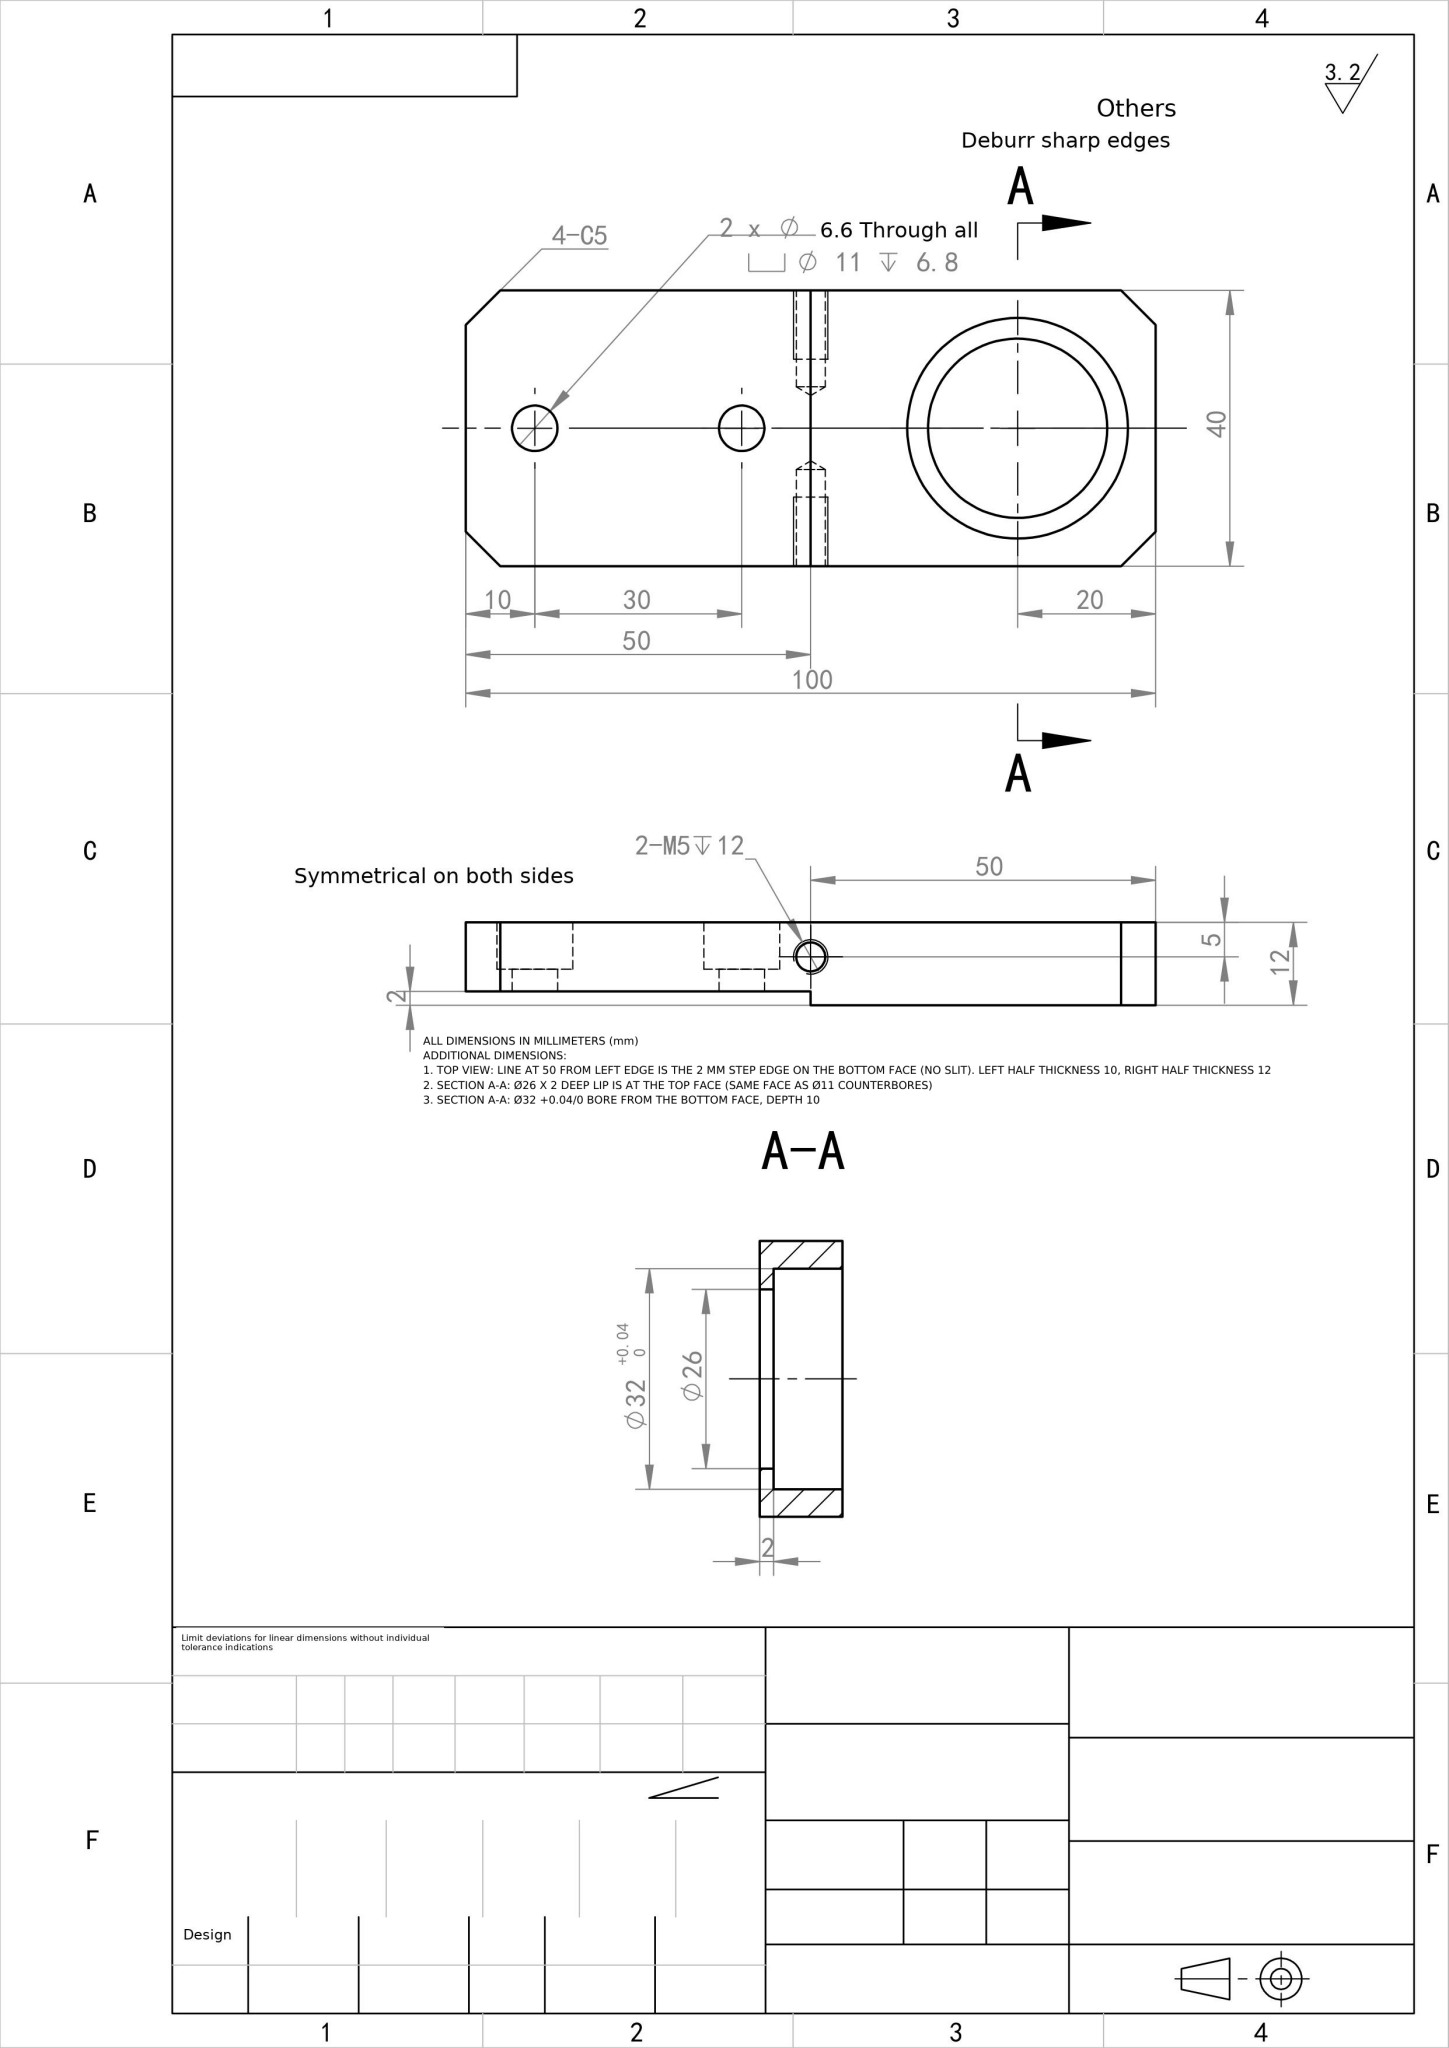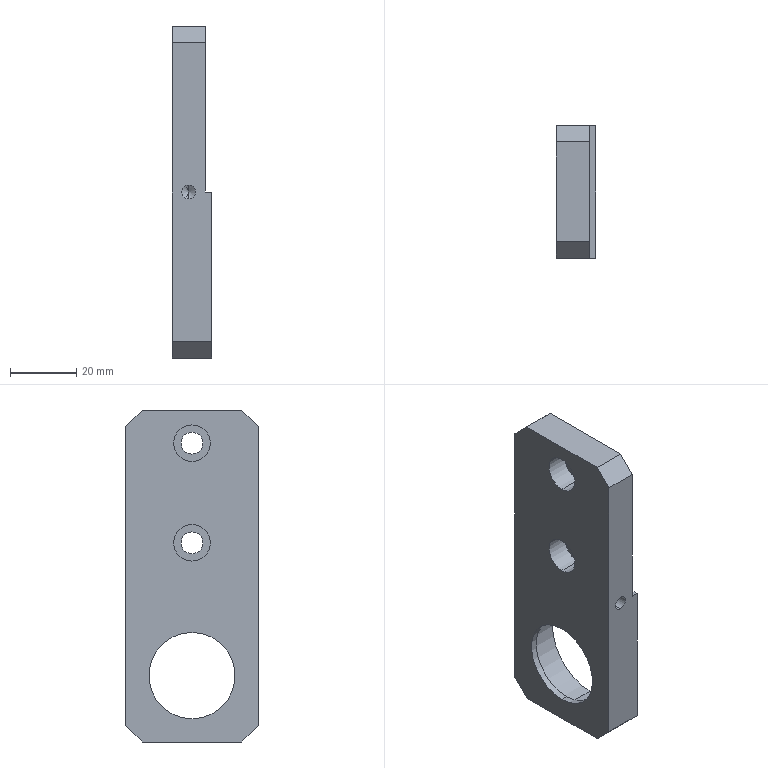Part | NX | mm | 1 solid | 35 faces | box 12 x 40 x 100 mm | volume 32435 mm3 | cylinder 16 | plane 15 | cone 4 | commonest cylinder face diameters 4.2 x4 11 x4 6.6 x4 26 x2 32 x2